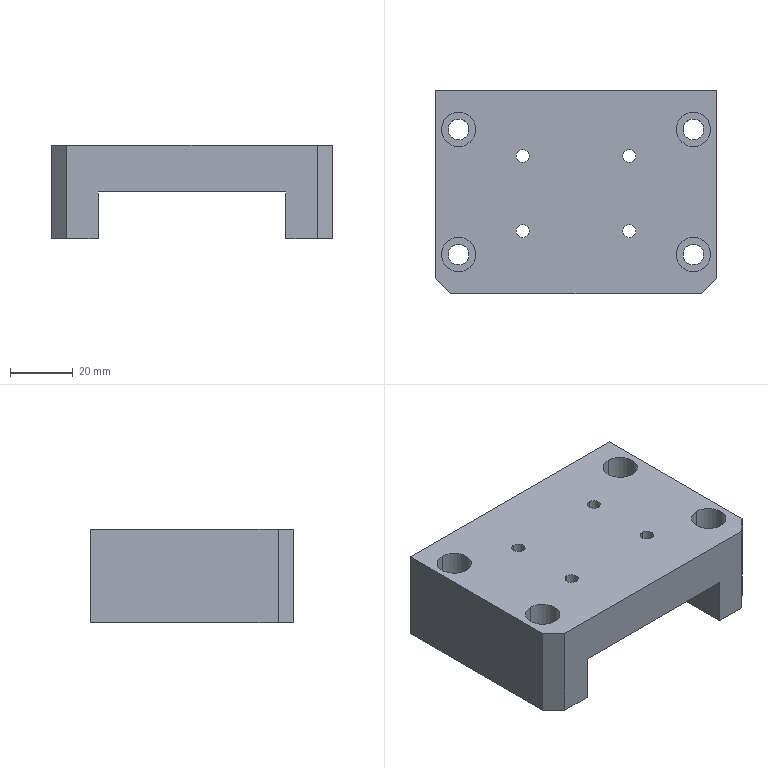Component | SolidWorks | RetractableStop-LongSide-1_CylinderConnectionPlate-LongSide-0510-1 | 1 solid | 40 faces | box 90 x 65 x 30 mm | volume 106448 mm3 | cylinder 24 | plane 16 | commonest cylinder face diameters 4.2 x8 11 x8 6.6 x8 | material Q235-A
build123d program:
from build123d import *

# Parameters (mm, degrees)
BOSS_EXTRUDE1_DEPTH                                = 65
HOLE_SIZE_ACCORDING_TO_TYPE_OF_HEX_SOC_D           = 6.6
HOLE_SIZE_ACCORDING_TO_TYPE_OF_HEX_SOC_CBORE_D     = 11
HOLE_SIZE_ACCORDING_TO_TYPE_OF_HEX_SOC_CBORE_DEPTH = 20
M5_TAPPED_HOLE1_D                                  = 4.2
CHAMFER2_SIZE                                      = 5


with BuildPart() as part:
    # Sketch1 → Boss-Extrude1 (new body)
    with BuildSketch(Plane.XY):
        Polygon((0, 0), (0, -30), (90, -30), (90, 0), (75, 0), (75, -15), (15, -15), (15, 0), align=None)
    extrude(amount=BOSS_EXTRUDE1_DEPTH)

    # Hole Size _According to_ Type of Hex Soc (through all)
    with Locations(Plane(origin=(0, -30, 0), x_dir=(-1, 0, 0), z_dir=(0, -1, 0))):
        with Locations((-7.5, -52.5), (-7.5, -12.5), (-82.5, -12.5), (-82.5, -52.5)):
            CounterBoreHole(HOLE_SIZE_ACCORDING_TO_TYPE_OF_HEX_SOC_D / 2, HOLE_SIZE_ACCORDING_TO_TYPE_OF_HEX_SOC_CBORE_D / 2, HOLE_SIZE_ACCORDING_TO_TYPE_OF_HEX_SOC_CBORE_DEPTH)

    # M5 Tapped Hole1 (through all)
    with Locations(Plane(origin=(0, -15, 0), x_dir=(1, 0, 0), z_dir=(0, 1, 0))):
        with Locations((28, -21), (28, -45), (62, -45), (62, -21)):
            Hole(M5_TAPPED_HOLE1_D / 2)

    # Chamfer2
    chamfer2_edges = [part.edges().sort_by_distance(p)[0] for p in [
        (90, -15, 65),
        (0, -15, 65),
    ]]
    chamfer(chamfer2_edges, length=CHAMFER2_SIZE)


solid = part.part

# Placed as in the assembly
solid = solid.moved(Location((-1287.013, 96.236, 3562.5), (90, 0, -180)))